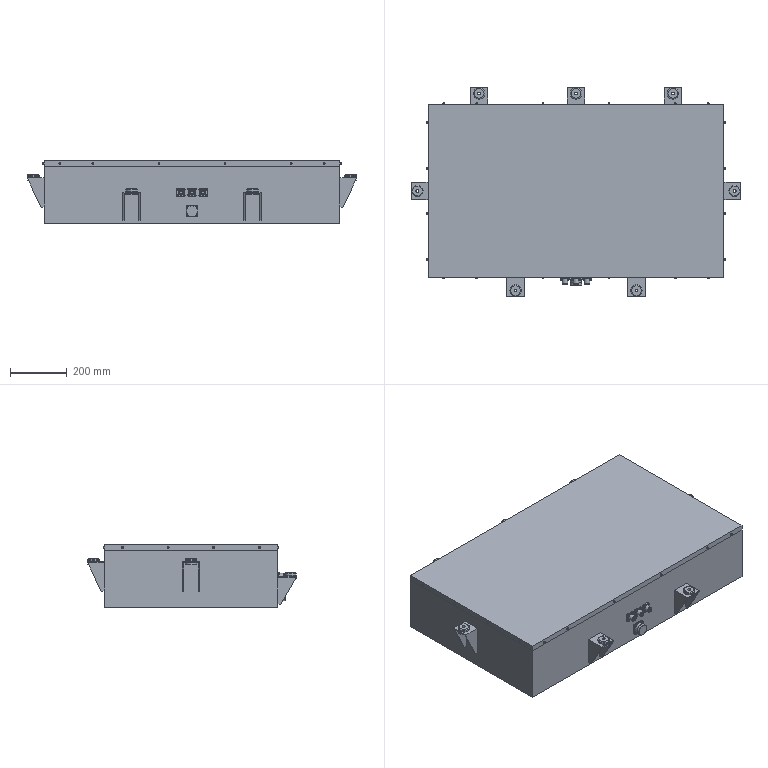Assembly | NX | mm | 49 component files | 49 solids | 1277 faces | box 1155 x 732.5 x 220 mm | volume 22857500 mm3 | plane 704 | cone 290 | cylinder 191 | torus 92 | commonest cylinder face diameters 3.838 x36 7 x36 4.5 x36 4 x36 40 x15 25 x14 10.2 x7 22.2 x3
Bill of materials:
unnamed part 1 | 3 |  | Thin square flange plate with four corner holes and a cylindrical tubular boss projecting from one face; the boss has a central bore and a rounded (filleted) outer edge at its free end.
unnamed part 2 | 7 |  | Axisymmetric spool-shaped part: an upper disc with rounded edges and a lower disc with sharp edges, joined by a narrower cylindrical neck that forms a circumferential groove, with a central through hole.
unnamed part 3 | 1 |  | Thin, flat rectangular plate with plain faces and small holes drilled into its edge faces.
unnamed part 4 | 1 |  | Open-top rectangular box or tray with a stepped rim around the top edge, mounting tabs with holes around the outside, and a group of holes in one side wall.
unnamed part 5 | 1 |  | Square flange plate with four corner holes and a solid cylindrical body projecting from one face, ending in a larger-diameter collar with chamfered edges and a flat, closed end face.
GB-T70.1-2000,M4x12 | 36 |  | Hexagon Socket Head Cap Screw, GB-T 70.1-2000,M4x12
Mates:
1. concentric | top_cover 1 edge | enclosure 1 edge
2. fix | enclosure 1 component
3. concentric | rubber_pad 7 edge | enclosure 1 edge
4. concentric | rubber_pad 6 edge | enclosure 1 edge
5. concentric | rubber_pad 5 edge | enclosure 1 edge
6. concentric | rubber_pad 4 edge | enclosure 1 edge
7. concentric | rubber_pad 3 edge | enclosure 1 edge
8. concentric | rubber_pad 2 edge | enclosure 1 edge
9. concentric | rubber_pad 1 edge | enclosure 1 edge
10. concentric | interface 3 edge | enclosure 1 edge
11. fix | assembly component
12. bond | interface 3 component | assembly component
13. bond | interface 2 component | assembly component
14. linear | assembly datumaxis | assembly cartesiancoordinatesystem | assembly cartesiancoordinatesystem | assembly cartesiancoordinatesystem
15. bond | interface 1 component | assembly component
16. concentric | button 1 edge | enclosure 1 edge
17. bond | interface 3 component | assembly component
18. bond | GB-T70_1-2000_M4x12 36 component | assembly component
19. bond | GB-T70_1-2000_M4x12 35 component | assembly component
20. bond | GB-T70_1-2000_M4x12 34 component | assembly component
21. bond | GB-T70_1-2000_M4x12 33 component | assembly component
22. circular | assembly datumaxis | assembly cartesiancoordinatesystem | assembly cartesiancoordinatesystem | assembly cartesiancoordinatesystem | assembly cartesiancoordinatesystem
23. bond | GB-T70_1-2000_M4x12 36 component | assembly component
24. bond | GB-T70_1-2000_M4x12 32 component | assembly component
25. bond | GB-T70_1-2000_M4x12 31 component | assembly component
26. linear | assembly datumaxis | assembly cartesiancoordinatesystem | assembly cartesiancoordinatesystem | assembly cartesiancoordinatesystem
27. bond | GB-T70_1-2000_M4x12 35 component | assembly component
28. bond | GB-T70_1-2000_M4x12 30 component | assembly component
29. bond | GB-T70_1-2000_M4x12 29 component | assembly component
30. linear | assembly datumaxis | assembly cartesiancoordinatesystem | assembly cartesiancoordinatesystem | assembly cartesiancoordinatesystem
31. bond | GB-T70_1-2000_M4x12 33 component | assembly component
32. bond | GB-T70_1-2000_M4x12 28 component | assembly component
33. bond | GB-T70_1-2000_M4x12 27 component | assembly component
34. linear | assembly datumaxis | assembly cartesiancoordinatesystem | assembly cartesiancoordinatesystem | assembly cartesiancoordinatesystem
35. bond | GB-T70_1-2000_M4x12 34 component | assembly component
36. bond | GB-T70_1-2000_M4x12 26 component | assembly component
37. bond | GB-T70_1-2000_M4x12 25 component | assembly component
38. linear | assembly datumaxis | assembly cartesiancoordinatesystem | assembly cartesiancoordinatesystem | assembly cartesiancoordinatesystem
39. bond | button 1 component | assembly component
40. bond | GB-T70_1-2000_M4x12 24 component | assembly component
41. bond | GB-T70_1-2000_M4x12 23 component | assembly component
42. bond | GB-T70_1-2000_M4x12 22 component | assembly component
43. bond | GB-T70_1-2000_M4x12 21 component | assembly component
44. circular | assembly datumaxis | assembly cartesiancoordinatesystem | assembly cartesiancoordinatesystem | assembly cartesiancoordinatesystem | assembly cartesiancoordinatesystem